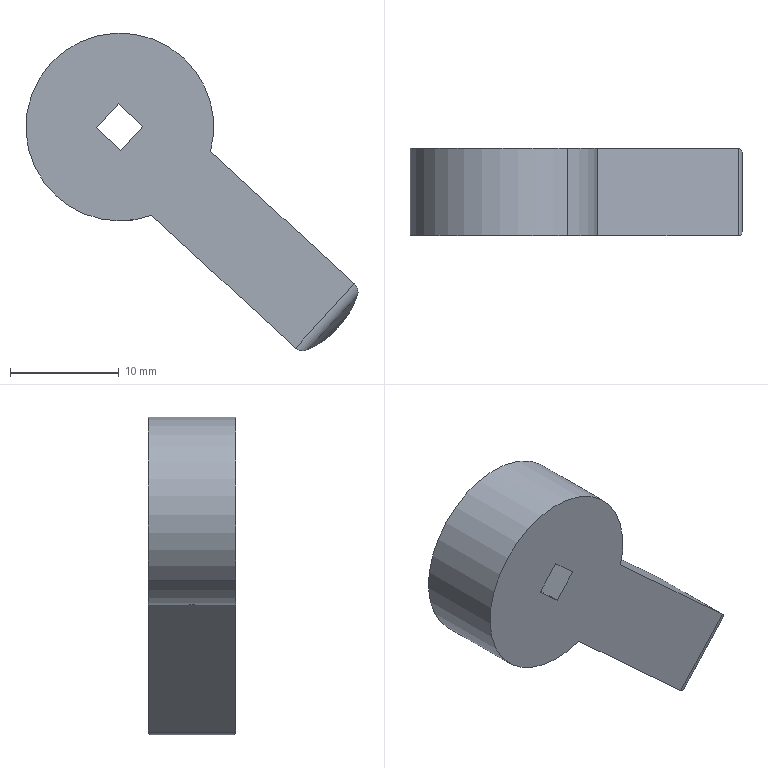Component | SolidWorks | Poussoir-1 | 1 solid | 24 faces | box 30.51 x 8 x 29.19 mm | volume 2976 mm3 | cylinder 11 | plane 9 | spline 4 | commonest cylinder face diameters 17 x4 2 x4 17.25 x3
STEP:
#1=CARTESIAN_POINT('',(2.86,2.961,-1.549));
#2=VERTEX_POINT('',#1);
#3=CARTESIAN_POINT('',(2.958,2.961,-1.887));
#4=VERTEX_POINT('',#3);
#5=CARTESIAN_POINT('',(2.63,2.961,-1.799));
#6=DIRECTION('',(0.,1.,-0.));
#7=DIRECTION('',(0.6774,0.,0.7356));
#8=AXIS2_PLACEMENT_3D('',#5,#6,#7);
#9=CIRCLE('',#8,0.3396);
#10=EDGE_CURVE('',#2,#4,#9,.T.);
#11=ORIENTED_EDGE('',*,*,#10,.F.);
#12=CARTESIAN_POINT('',(2.86,2.646,-1.549));
#13=VERTEX_POINT('',#12);
#14=CARTESIAN_POINT('',(2.86,2.961,-1.549));
#15=DIRECTION('',(-0.,-1.,0.));
#16=VECTOR('',#15,39.37);
#17=LINE('',#14,#16);
#18=EDGE_CURVE('',#2,#13,#17,.T.);
#19=ORIENTED_EDGE('',*,*,#18,.T.);
#20=CARTESIAN_POINT('',(2.958,2.646,-1.887));
#21=VERTEX_POINT('',#20);
#22=CARTESIAN_POINT('',(2.63,2.646,-1.799));
#23=DIRECTION('',(0.,1.,-0.));
#24=DIRECTION('',(0.6774,0.,0.7356));
#25=AXIS2_PLACEMENT_3D('',#22,#23,#24);
#26=CIRCLE('',#25,0.3396);
#27=EDGE_CURVE('',#13,#21,#26,.T.);
#28=ORIENTED_EDGE('',*,*,#27,.T.);
#29=CARTESIAN_POINT('',(2.958,2.961,-1.887));
#30=DIRECTION('',(-0.,-1.,0.));
#31=VECTOR('',#30,39.37);
#32=LINE('',#29,#31);
#33=EDGE_CURVE('',#4,#21,#32,.T.);
#34=ORIENTED_EDGE('',*,*,#33,.F.);
#35=EDGE_LOOP('',(#11,#19,#28,#34));
#36=FACE_OUTER_BOUND('',#35,.T.);
#37=CARTESIAN_POINT('',(2.63,2.961,-1.799));
#38=DIRECTION('',(-0.,-1.,0.));
#39=DIRECTION('',(-0.6774,0.,-0.7356));
#40=AXIS2_PLACEMENT_3D('',#37,#38,#39);
#41=CYLINDRICAL_SURFACE('',#40,0.3396);
#42=ADVANCED_FACE('',(#36),#41,.T.);
#43=ORIENTED_EDGE('',*,*,#18,.F.);
#44=CARTESIAN_POINT('',(2.4,2.961,-2.049));
#45=VERTEX_POINT('',#44);
#46=CARTESIAN_POINT('',(2.63,2.961,-1.799));
#47=DIRECTION('',(0.,1.,-0.));
#48=DIRECTION('',(0.6774,0.,0.7356));
#49=AXIS2_PLACEMENT_3D('',#46,#47,#48);
#50=CIRCLE('',#49,0.3396);
#51=EDGE_CURVE('',#45,#2,#50,.T.);
#52=ORIENTED_EDGE('',*,*,#51,.F.);
#53=CARTESIAN_POINT('',(2.4,2.646,-2.049));
#54=VERTEX_POINT('',#53);
#55=CARTESIAN_POINT('',(2.4,2.961,-2.049));
#56=DIRECTION('',(-0.,-1.,0.));
#57=VECTOR('',#56,39.37);
#58=LINE('',#55,#57);
#59=EDGE_CURVE('',#45,#54,#58,.T.);
#60=ORIENTED_EDGE('',*,*,#59,.T.);
#61=CARTESIAN_POINT('',(2.63,2.646,-1.799));
#62=DIRECTION('',(0.,1.,-0.));
#63=DIRECTION('',(0.6774,0.,0.7356));
#64=AXIS2_PLACEMENT_3D('',#61,#62,#63);
#65=CIRCLE('',#64,0.3396);
#66=EDGE_CURVE('',#54,#13,#65,.T.);
#67=ORIENTED_EDGE('',*,*,#66,.T.);
#68=EDGE_LOOP('',(#43,#52,#60,#67));
#69=FACE_OUTER_BOUND('',#68,.T.);
#70=CARTESIAN_POINT('',(2.63,2.961,-1.799));
#71=DIRECTION('',(-0.,-1.,0.));
#72=DIRECTION('',(-0.6774,0.,-0.7356));
#73=AXIS2_PLACEMENT_3D('',#70,#71,#72);
#74=CYLINDRICAL_SURFACE('',#73,0.3396);
#75=ADVANCED_FACE('',(#69),#74,.T.);
#76=CARTESIAN_POINT('',(3.419,2.803,-2.526));
#77=VERTEX_POINT('',#76);
#78=CARTESIAN_POINT('',(3.308,2.669,-2.605));
#79=VERTEX_POINT('',#78);
#80=CARTESIAN_POINT('',(3.419,2.803,-2.526));
#81=CARTESIAN_POINT('',(3.388,2.757,-2.56));
#82=CARTESIAN_POINT('',(3.35,2.712,-2.586));
#83=CARTESIAN_POINT('',(3.308,2.669,-2.605));
#84=(BOUNDED_CURVE()B_SPLINE_CURVE(3,(#80,#81,#82,#83),.UNSPECIFIED.,.F.,.F.)B_SPLINE_CURVE_WITH_KNOTS((4,4),(1.571,1.982),.UNSPECIFIED.)CURVE()GEOMETRIC_REPRESENTATION_ITEM()RATIONAL_B_SPLINE_CURVE((1.,0.9859,0.9859,1.))REPRESENTATION_ITEM(''));
#85=EDGE_CURVE('',#77,#79,#84,.T.);
#86=ORIENTED_EDGE('',*,*,#85,.T.);
#87=CARTESIAN_POINT('',(3.308,2.937,-2.605));
#88=VERTEX_POINT('',#87);
#89=CARTESIAN_POINT('',(3.308,2.646,-2.605));
#90=DIRECTION('',(0.,1.,-0.));
#91=VECTOR('',#90,39.37);
#92=LINE('',#89,#91);
#93=EDGE_CURVE('',#79,#88,#92,.T.);
#94=ORIENTED_EDGE('',*,*,#93,.T.);
#95=CARTESIAN_POINT('',(3.308,2.937,-2.605));
#96=CARTESIAN_POINT('',(3.35,2.895,-2.586));
#97=CARTESIAN_POINT('',(3.388,2.849,-2.56));
#98=CARTESIAN_POINT('',(3.419,2.803,-2.526));
#99=(BOUNDED_CURVE()B_SPLINE_CURVE(3,(#95,#96,#97,#98),.UNSPECIFIED.,.F.,.F.)B_SPLINE_CURVE_WITH_KNOTS((4,4),(1.159,1.571),.UNSPECIFIED.)CURVE()GEOMETRIC_REPRESENTATION_ITEM()RATIONAL_B_SPLINE_CURVE((1.,0.9859,0.9859,1.))REPRESENTATION_ITEM(''));
#100=EDGE_CURVE('',#88,#77,#99,.T.);
#101=ORIENTED_EDGE('',*,*,#100,.T.);
#102=EDGE_LOOP('',(#86,#94,#101));
#103=FACE_OUTER_BOUND('',#102,.T.);
#104=CARTESIAN_POINT('',(3.173,2.646,-2.299));
#105=DIRECTION('',(0.,1.,-0.));
#106=DIRECTION('',(0.6774,0.,0.7356));
#107=AXIS2_PLACEMENT_3D('',#104,#105,#106);
#108=CYLINDRICAL_SURFACE('',#107,0.3346);
#109=ADVANCED_FACE('',(#103),#108,.T.);
#110=CARTESIAN_POINT('',(3.479,2.961,-2.366));
#111=VERTEX_POINT('',#110);
#112=CARTESIAN_POINT('',(3.526,2.961,-2.41));
#113=DIRECTION('',(0.7356,-0.,-0.6774));
#114=VECTOR('',#113,39.37);
#115=LINE('',#112,#114);
#116=EDGE_CURVE('',#4,#111,#115,.T.);
#117=ORIENTED_EDGE('',*,*,#116,.T.);
#118=CARTESIAN_POINT('',(3.266,2.961,-2.598));
#119=VERTEX_POINT('',#118);
#120=CARTESIAN_POINT('',(3.266,2.961,-2.598));
#121=DIRECTION('',(-0.6774,0.,-0.7356));
#122=VECTOR('',#121,39.37);
#123=LINE('',#120,#122);
#124=EDGE_CURVE('',#111,#119,#123,.T.);
#125=ORIENTED_EDGE('',*,*,#124,.T.);
#126=CARTESIAN_POINT('',(2.745,2.961,-2.118));
#127=VERTEX_POINT('',#126);
#128=CARTESIAN_POINT('',(3.313,2.961,-2.641));
#129=DIRECTION('',(-0.7356,0.,0.6774));
#130=VECTOR('',#129,39.37);
#131=LINE('',#128,#130);
#132=EDGE_CURVE('',#119,#127,#131,.T.);
#133=ORIENTED_EDGE('',*,*,#132,.T.);
#134=CARTESIAN_POINT('',(2.63,2.961,-1.799));
#135=DIRECTION('',(0.,1.,-0.));
#136=DIRECTION('',(0.6774,0.,0.7356));
#137=AXIS2_PLACEMENT_3D('',#134,#135,#136);
#138=CIRCLE('',#137,0.3396);
#139=EDGE_CURVE('',#127,#45,#138,.T.);
#140=ORIENTED_EDGE('',*,*,#139,.T.);
#141=ORIENTED_EDGE('',*,*,#51,.T.);
#142=ORIENTED_EDGE('',*,*,#10,.T.);
#143=EDGE_LOOP('',(#117,#125,#133,#140,#141,#142));
#144=FACE_OUTER_BOUND('',#143,.T.);
#145=CARTESIAN_POINT('',(2.547,2.961,-1.802));
#146=VERTEX_POINT('',#145);
#147=CARTESIAN_POINT('',(2.627,2.961,-1.715));
#148=VERTEX_POINT('',#147);
#149=CARTESIAN_POINT('',(2.627,2.961,-1.715));
#150=DIRECTION('',(0.6774,-0.,0.7356));
#151=VECTOR('',#150,39.37);
#152=LINE('',#149,#151);
#153=EDGE_CURVE('',#146,#148,#152,.T.);
#154=ORIENTED_EDGE('',*,*,#153,.F.);
#155=CARTESIAN_POINT('',(2.634,2.961,-1.882));
#156=VERTEX_POINT('',#155);
#157=CARTESIAN_POINT('',(2.547,2.961,-1.802));
#158=DIRECTION('',(-0.7356,0.,0.6774));
#159=VECTOR('',#158,39.37);
#160=LINE('',#157,#159);
#161=EDGE_CURVE('',#156,#146,#160,.T.);
#162=ORIENTED_EDGE('',*,*,#161,.F.);
#163=CARTESIAN_POINT('',(2.714,2.961,-1.795));
#164=VERTEX_POINT('',#163);
#165=CARTESIAN_POINT('',(2.714,2.961,-1.795));
#166=DIRECTION('',(-0.6774,0.,-0.7356));
#167=VECTOR('',#166,39.37);
#168=LINE('',#165,#167);
#169=EDGE_CURVE('',#164,#156,#168,.T.);
#170=ORIENTED_EDGE('',*,*,#169,.F.);
#171=CARTESIAN_POINT('',(2.627,2.961,-1.715));
#172=DIRECTION('',(0.7356,-0.,-0.6774));
#173=VECTOR('',#172,39.37);
#174=LINE('',#171,#173);
#175=EDGE_CURVE('',#148,#164,#174,.T.);
#176=ORIENTED_EDGE('',*,*,#175,.F.);
#177=EDGE_LOOP('',(#154,#162,#170,#176));
#178=FACE_BOUND('',#177,.T.);
#179=CARTESIAN_POINT('',(2.63,2.961,-1.799));
#180=DIRECTION('',(0.,1.,-0.));
#181=DIRECTION('',(0.6774,-0.,0.7356));
#182=AXIS2_PLACEMENT_3D('',#179,#180,#181);
#183=PLANE('',#182);
#184=ADVANCED_FACE('',(#144,#178),#183,.T.);
#185=CARTESIAN_POINT('',(3.266,2.646,-2.598));
#186=VERTEX_POINT('',#185);
#187=CARTESIAN_POINT('',(2.745,2.646,-2.118));
#188=VERTEX_POINT('',#187);
#189=CARTESIAN_POINT('',(3.313,2.646,-2.641));
#190=DIRECTION('',(-0.7356,0.,0.6774));
#191=VECTOR('',#190,39.37);
#192=LINE('',#189,#191);
#193=EDGE_CURVE('',#186,#188,#192,.T.);
#194=ORIENTED_EDGE('',*,*,#193,.F.);
#195=CARTESIAN_POINT('',(3.479,2.646,-2.366));
#196=VERTEX_POINT('',#195);
#197=CARTESIAN_POINT('',(3.372,2.646,-2.482));
#198=DIRECTION('',(0.6774,-0.,0.7356));
#199=VECTOR('',#198,39.37);
#200=LINE('',#197,#199);
#201=EDGE_CURVE('',#186,#196,#200,.T.);
#202=ORIENTED_EDGE('',*,*,#201,.T.);
#203=CARTESIAN_POINT('',(3.526,2.646,-2.41));
#204=DIRECTION('',(0.7356,-0.,-0.6774));
#205=VECTOR('',#204,39.37);
#206=LINE('',#203,#205);
#207=EDGE_CURVE('',#21,#196,#206,.T.);
#208=ORIENTED_EDGE('',*,*,#207,.F.);
#209=ORIENTED_EDGE('',*,*,#27,.F.);
#210=ORIENTED_EDGE('',*,*,#66,.F.);
#211=CARTESIAN_POINT('',(2.63,2.646,-1.799));
#212=DIRECTION('',(0.,1.,-0.));
#213=DIRECTION('',(0.6774,0.,0.7356));
#214=AXIS2_PLACEMENT_3D('',#211,#212,#213);
#215=CIRCLE('',#214,0.3396);
#216=EDGE_CURVE('',#188,#54,#215,.T.);
#217=ORIENTED_EDGE('',*,*,#216,.F.);
#218=EDGE_LOOP('',(#194,#202,#208,#209,#210,#217));
#219=FACE_OUTER_BOUND('',#218,.T.);
#220=CARTESIAN_POINT('',(2.634,2.646,-1.882));
#221=VERTEX_POINT('',#220);
#222=CARTESIAN_POINT('',(2.547,2.646,-1.802));
#223=VERTEX_POINT('',#222);
#224=CARTESIAN_POINT('',(2.547,2.646,-1.802));
#225=DIRECTION('',(-0.7356,0.,0.6774));
#226=VECTOR('',#225,39.37);
#227=LINE('',#224,#226);
#228=EDGE_CURVE('',#221,#223,#227,.T.);
#229=ORIENTED_EDGE('',*,*,#228,.T.);
#230=CARTESIAN_POINT('',(2.627,2.646,-1.715));
#231=VERTEX_POINT('',#230);
#232=CARTESIAN_POINT('',(2.627,2.646,-1.715));
#233=DIRECTION('',(0.6774,-0.,0.7356));
#234=VECTOR('',#233,39.37);
#235=LINE('',#232,#234);
#236=EDGE_CURVE('',#223,#231,#235,.T.);
#237=ORIENTED_EDGE('',*,*,#236,.T.);
#238=CARTESIAN_POINT('',(2.714,2.646,-1.795));
#239=VERTEX_POINT('',#238);
#240=CARTESIAN_POINT('',(2.627,2.646,-1.715));
#241=DIRECTION('',(0.7356,-0.,-0.6774));
#242=VECTOR('',#241,39.37);
#243=LINE('',#240,#242);
#244=EDGE_CURVE('',#231,#239,#243,.T.);
#245=ORIENTED_EDGE('',*,*,#244,.T.);
#246=CARTESIAN_POINT('',(2.714,2.646,-1.795));
#247=DIRECTION('',(-0.6774,0.,-0.7356));
#248=VECTOR('',#247,39.37);
#249=LINE('',#246,#248);
#250=EDGE_CURVE('',#239,#221,#249,.T.);
#251=ORIENTED_EDGE('',*,*,#250,.T.);
#252=EDGE_LOOP('',(#229,#237,#245,#251));
#253=FACE_BOUND('',#252,.T.);
#254=CARTESIAN_POINT('',(2.63,2.646,-1.799));
#255=DIRECTION('',(0.,1.,-0.));
#256=DIRECTION('',(0.6774,-0.,0.7356));
#257=AXIS2_PLACEMENT_3D('',#254,#255,#256);
#258=PLANE('',#257);
#259=ADVANCED_FACE('',(#219,#253),#258,.F.);
#260=ORIENTED_EDGE('',*,*,#132,.F.);
#261=CARTESIAN_POINT('',(3.266,2.961,-2.598));
#262=DIRECTION('',(-0.,-1.,0.));
#263=VECTOR('',#262,39.37);
#264=LINE('',#261,#263);
#265=EDGE_CURVE('',#119,#186,#264,.T.);
#266=ORIENTED_EDGE('',*,*,#265,.T.);
#267=ORIENTED_EDGE('',*,*,#193,.T.);
#268=CARTESIAN_POINT('',(2.745,2.961,-2.118));
#269=DIRECTION('',(-0.,-1.,0.));
#270=VECTOR('',#269,39.37);
#271=LINE('',#268,#270);
#272=EDGE_CURVE('',#127,#188,#271,.T.);
#273=ORIENTED_EDGE('',*,*,#272,.F.);
#274=EDGE_LOOP('',(#260,#266,#267,#273));
#275=FACE_OUTER_BOUND('',#274,.T.);
#276=CARTESIAN_POINT('',(3.313,2.961,-2.641));
#277=DIRECTION('',(0.6774,-0.,0.7356));
#278=DIRECTION('',(0.7356,-0.,-0.6774));
#279=AXIS2_PLACEMENT_3D('',#276,#277,#278);
#280=PLANE('',#279);
#281=ADVANCED_FACE('',(#275),#280,.F.);
#282=ORIENTED_EDGE('',*,*,#59,.F.);
#283=ORIENTED_EDGE('',*,*,#139,.F.);
#284=ORIENTED_EDGE('',*,*,#272,.T.);
#285=ORIENTED_EDGE('',*,*,#216,.T.);
#286=EDGE_LOOP('',(#282,#283,#284,#285));
#287=FACE_OUTER_BOUND('',#286,.T.);
#288=CARTESIAN_POINT('',(2.605,2.803,-2.137));
#289=VERTEX_POINT('',#288);
#290=CARTESIAN_POINT('',(2.644,2.764,-2.138));
#291=VERTEX_POINT('',#290);
#292=CARTESIAN_POINT('',(2.605,2.803,-2.137));
#293=CARTESIAN_POINT('',(2.605,2.798,-2.137));
#294=CARTESIAN_POINT('',(2.606,2.793,-2.137));
#295=CARTESIAN_POINT('',(2.61,2.783,-2.138));
#296=CARTESIAN_POINT('',(2.613,2.779,-2.138));
#297=CARTESIAN_POINT('',(2.623,2.768,-2.138));
#298=CARTESIAN_POINT('',(2.634,2.764,-2.138));
#299=CARTESIAN_POINT('',(2.644,2.764,-2.138));
#300=B_SPLINE_CURVE_WITH_KNOTS('',3,(#292,#293,#294,#295,#296,#297,#298,#299),.UNSPECIFIED.,.F.,.F.,(4,2,2,4),(0.,0.0003909,0.0007817,0.001563),.UNSPECIFIED.);
#301=EDGE_CURVE('',#289,#291,#300,.T.);
#302=ORIENTED_EDGE('',*,*,#301,.T.);
#303=CARTESIAN_POINT('',(2.683,2.803,-2.134));
#304=VERTEX_POINT('',#303);
#305=CARTESIAN_POINT('',(2.644,2.764,-2.138));
#306=CARTESIAN_POINT('',(2.649,2.764,-2.138));
#307=CARTESIAN_POINT('',(2.654,2.765,-2.137));
#308=CARTESIAN_POINT('',(2.664,2.769,-2.137));
#309=CARTESIAN_POINT('',(2.668,2.772,-2.136));
#310=CARTESIAN_POINT('',(2.679,2.783,-2.135));
#311=CARTESIAN_POINT('',(2.683,2.793,-2.134));
#312=CARTESIAN_POINT('',(2.683,2.803,-2.134));
#313=B_SPLINE_CURVE_WITH_KNOTS('',3,(#305,#306,#307,#308,#309,#310,#311,#312),.UNSPECIFIED.,.F.,.F.,(4,2,2,4),(0.,0.0003909,0.0007817,0.001563),.UNSPECIFIED.);
#314=EDGE_CURVE('',#291,#304,#313,.T.);
#315=ORIENTED_EDGE('',*,*,#314,.T.);
#316=CARTESIAN_POINT('',(2.644,2.843,-2.138));
#317=VERTEX_POINT('',#316);
#318=CARTESIAN_POINT('',(2.683,2.803,-2.134));
#319=CARTESIAN_POINT('',(2.683,2.808,-2.134));
#320=CARTESIAN_POINT('',(2.682,2.813,-2.134));
#321=CARTESIAN_POINT('',(2.678,2.823,-2.135));
#322=CARTESIAN_POINT('',(2.675,2.827,-2.135));
#323=CARTESIAN_POINT('',(2.665,2.838,-2.137));
#324=CARTESIAN_POINT('',(2.654,2.843,-2.138));
#325=CARTESIAN_POINT('',(2.644,2.843,-2.138));
#326=B_SPLINE_CURVE_WITH_KNOTS('',3,(#318,#319,#320,#321,#322,#323,#324,#325),.UNSPECIFIED.,.F.,.F.,(4,2,2,4),(0.,0.0003909,0.0007817,0.001563),.UNSPECIFIED.);
#327=EDGE_CURVE('',#304,#317,#326,.T.);
#328=ORIENTED_EDGE('',*,*,#327,.T.);
#329=CARTESIAN_POINT('',(2.644,2.843,-2.138));
#330=CARTESIAN_POINT('',(2.639,2.843,-2.138));
#331=CARTESIAN_POINT('',(2.634,2.841,-2.138));
#332=CARTESIAN_POINT('',(2.624,2.838,-2.138));
#333=CARTESIAN_POINT('',(2.62,2.835,-2.138));
#334=CARTESIAN_POINT('',(2.609,2.824,-2.138));
#335=CARTESIAN_POINT('',(2.605,2.814,-2.137));
#336=CARTESIAN_POINT('',(2.605,2.803,-2.137));
#337=B_SPLINE_CURVE_WITH_KNOTS('',3,(#329,#330,#331,#332,#333,#334,#335,#336),.UNSPECIFIED.,.F.,.F.,(4,2,2,4),(0.,0.0003909,0.0007817,0.001563),.UNSPECIFIED.);
#338=EDGE_CURVE('',#317,#289,#337,.T.);
#339=ORIENTED_EDGE('',*,*,#338,.T.);
#340=EDGE_LOOP('',(#302,#315,#328,#339));
#341=FACE_BOUND('',#340,.T.);
#342=CARTESIAN_POINT('',(2.63,2.961,-1.799));
#343=DIRECTION('',(-0.,-1.,0.));
#344=DIRECTION('',(-0.6774,0.,-0.7356));
#345=AXIS2_PLACEMENT_3D('',#342,#343,#344);
#346=CYLINDRICAL_SURFACE('',#345,0.3396);
#347=ADVANCED_FACE('',(#287,#341),#346,.T.);
#348=ORIENTED_EDGE('',*,*,#207,.T.);
#349=CARTESIAN_POINT('',(3.479,2.961,-2.366));
#350=DIRECTION('',(0.,1.,-0.));
#351=VECTOR('',#350,39.37);
#352=LINE('',#349,#351);
#353=EDGE_CURVE('',#196,#111,#352,.T.);
#354=ORIENTED_EDGE('',*,*,#353,.T.);
#355=ORIENTED_EDGE('',*,*,#116,.F.);
#356=ORIENTED_EDGE('',*,*,#33,.T.);
#357=EDGE_LOOP('',(#348,#354,#355,#356));
#358=FACE_OUTER_BOUND('',#357,.T.);
#359=CARTESIAN_POINT('',(3.526,2.961,-2.41));
#360=DIRECTION('',(-0.6774,0.,-0.7356));
#361=DIRECTION('',(-0.7356,0.,0.6774));
#362=AXIS2_PLACEMENT_3D('',#359,#360,#361);
#363=PLANE('',#362);
#364=ADVANCED_FACE('',(#358),#363,.F.);
#365=ORIENTED_EDGE('',*,*,#228,.F.);
#366=CARTESIAN_POINT('',(2.634,2.961,-1.882));
#367=DIRECTION('',(-0.,-1.,0.));
#368=VECTOR('',#367,39.37);
#369=LINE('',#366,#368);
#370=EDGE_CURVE('',#156,#221,#369,.T.);
#371=ORIENTED_EDGE('',*,*,#370,.F.);
#372=ORIENTED_EDGE('',*,*,#161,.T.);
#373=CARTESIAN_POINT('',(2.547,2.961,-1.802));
#374=DIRECTION('',(-0.,-1.,0.));
#375=VECTOR('',#374,39.37);
#376=LINE('',#373,#375);
#377=EDGE_CURVE('',#146,#223,#376,.T.);
#378=ORIENTED_EDGE('',*,*,#377,.T.);
#379=EDGE_LOOP('',(#365,#371,#372,#378));
#380=FACE_OUTER_BOUND('',#379,.T.);
#381=CARTESIAN_POINT('',(2.547,2.961,-1.802));
#382=DIRECTION('',(0.6774,-0.,0.7356));
#383=DIRECTION('',(-0.,-1.,0.));
#384=AXIS2_PLACEMENT_3D('',#381,#382,#383);
#385=PLANE('',#384);
#386=ADVANCED_FACE('',(#380),#385,.T.);
#387=ORIENTED_EDGE('',*,*,#236,.F.);
#388=ORIENTED_EDGE('',*,*,#377,.F.);
#389=ORIENTED_EDGE('',*,*,#153,.T.);
#390=CARTESIAN_POINT('',(2.627,2.961,-1.715));
#391=DIRECTION('',(-0.,-1.,0.));
#392=VECTOR('',#391,39.37);
#393=LINE('',#390,#392);
#394=EDGE_CURVE('',#148,#231,#393,.T.);
#395=ORIENTED_EDGE('',*,*,#394,.T.);
#396=EDGE_LOOP('',(#387,#388,#389,#395));
#397=FACE_OUTER_BOUND('',#396,.T.);
#398=CARTESIAN_POINT('',(2.627,2.961,-1.715));
#399=DIRECTION('',(0.7356,-0.,-0.6774));
#400=DIRECTION('',(-0.6774,0.,-0.7356));
#401=AXIS2_PLACEMENT_3D('',#398,#399,#400);
#402=PLANE('',#401);
#403=ADVANCED_FACE('',(#397),#402,.T.);
#404=ORIENTED_EDGE('',*,*,#244,.F.);
#405=ORIENTED_EDGE('',*,*,#394,.F.);
#406=ORIENTED_EDGE('',*,*,#175,.T.);
#407=CARTESIAN_POINT('',(2.714,2.961,-1.795));
#408=DIRECTION('',(-0.,-1.,0.));
#409=VECTOR('',#408,39.37);
#410=LINE('',#407,#409);
#411=EDGE_CURVE('',#164,#239,#410,.T.);
#412=ORIENTED_EDGE('',*,*,#411,.T.);
#413=EDGE_LOOP('',(#404,#405,#406,#412));
#414=FACE_OUTER_BOUND('',#413,.T.);
#415=CARTESIAN_POINT('',(2.627,2.961,-1.715));
#416=DIRECTION('',(-0.6774,0.,-0.7356));
#417=DIRECTION('',(0.,1.,-0.));
#418=AXIS2_PLACEMENT_3D('',#415,#416,#417);
#419=PLANE('',#418);
#420=ADVANCED_FACE('',(#414),#419,.T.);
#421=ORIENTED_EDGE('',*,*,#250,.F.);
#422=ORIENTED_EDGE('',*,*,#411,.F.);
#423=ORIENTED_EDGE('',*,*,#169,.T.);
#424=ORIENTED_EDGE('',*,*,#370,.T.);
#425=EDGE_LOOP('',(#421,#422,#423,#424));
#426=FACE_OUTER_BOUND('',#425,.T.);
#427=CARTESIAN_POINT('',(2.714,2.961,-1.795));
#428=DIRECTION('',(-0.7356,0.,0.6774));
#429=DIRECTION('',(0.6774,-0.,0.7356));
#430=AXIS2_PLACEMENT_3D('',#427,#428,#429);
#431=PLANE('',#430);
#432=ADVANCED_FACE('',(#426),#431,.T.);
#433=CARTESIAN_POINT('',(3.489,2.937,-2.408));
#434=VERTEX_POINT('',#433);
#435=CARTESIAN_POINT('',(3.419,2.803,-2.526));
#436=CARTESIAN_POINT('',(3.451,2.849,-2.492));
#437=CARTESIAN_POINT('',(3.474,2.895,-2.452));
#438=CARTESIAN_POINT('',(3.489,2.937,-2.408));
#439=(BOUNDED_CURVE()B_SPLINE_CURVE(3,(#435,#436,#437,#438),.UNSPECIFIED.,.F.,.F.)B_SPLINE_CURVE_WITH_KNOTS((4,4),(4.712,5.124),.UNSPECIFIED.)CURVE()GEOMETRIC_REPRESENTATION_ITEM()RATIONAL_B_SPLINE_CURVE((1.,0.9859,0.9859,1.))REPRESENTATION_ITEM(''));
#440=EDGE_CURVE('',#77,#434,#439,.T.);
#441=ORIENTED_EDGE('',*,*,#440,.T.);
#442=CARTESIAN_POINT('',(3.489,2.669,-2.408));
#443=VERTEX_POINT('',#442);
#444=CARTESIAN_POINT('',(3.489,2.646,-2.408));
#445=DIRECTION('',(-0.,-1.,0.));
#446=VECTOR('',#445,39.37);
#447=LINE('',#444,#446);
#448=EDGE_CURVE('',#434,#443,#447,.T.);
#449=ORIENTED_EDGE('',*,*,#448,.T.);
#450=CARTESIAN_POINT('',(3.489,2.669,-2.408));
#451=CARTESIAN_POINT('',(3.474,2.712,-2.452));
#452=CARTESIAN_POINT('',(3.451,2.757,-2.492));
#453=CARTESIAN_POINT('',(3.419,2.803,-2.526));
#454=(BOUNDED_CURVE()B_SPLINE_CURVE(3,(#450,#451,#452,#453),.UNSPECIFIED.,.F.,.F.)B_SPLINE_CURVE_WITH_KNOTS((4,4),(4.301,4.712),.UNSPECIFIED.)CURVE()GEOMETRIC_REPRESENTATION_ITEM()RATIONAL_B_SPLINE_CURVE((1.,0.9859,0.9859,1.))REPRESENTATION_ITEM(''));
#455=EDGE_CURVE('',#443,#77,#454,.T.);
#456=ORIENTED_EDGE('',*,*,#455,.T.);
#457=EDGE_LOOP('',(#441,#449,#456));
#458=FACE_OUTER_BOUND('',#457,.T.);
#459=CARTESIAN_POINT('',(3.173,2.646,-2.299));
#460=DIRECTION('',(0.,1.,-0.));
#461=DIRECTION('',(0.6774,0.,0.7356));
#462=AXIS2_PLACEMENT_3D('',#459,#460,#461);
#463=CYLINDRICAL_SURFACE('',#462,0.3346);
#464=ADVANCED_FACE('',(#458),#463,.T.);
#465=ORIENTED_EDGE('',*,*,#100,.F.);
#466=CARTESIAN_POINT('',(3.505,2.937,-2.391));
#467=DIRECTION('',(0.6774,-0.,0.7356));
#468=VECTOR('',#467,39.37);
#469=LINE('',#466,#468);
#470=EDGE_CURVE('',#88,#434,#469,.T.);
#471=ORIENTED_EDGE('',*,*,#470,.T.);
#472=ORIENTED_EDGE('',*,*,#440,.F.);
#473=EDGE_LOOP('',(#465,#471,#472));
#474=FACE_OUTER_BOUND('',#473,.T.);
#475=CARTESIAN_POINT('',(3.28,2.803,-2.183));
#476=DIRECTION('',(-0.6774,0.,-0.7356));
#477=DIRECTION('',(-0.7356,0.,0.6774));
#478=AXIS2_PLACEMENT_3D('',#475,#476,#477);
#479=CYLINDRICAL_SURFACE('',#478,0.3346);
#480=ADVANCED_FACE('',(#474),#479,.T.);
#481=ORIENTED_EDGE('',*,*,#455,.F.);
#482=CARTESIAN_POINT('',(3.505,2.669,-2.391));
#483=DIRECTION('',(-0.6774,0.,-0.7356));
#484=VECTOR('',#483,39.37);
#485=LINE('',#482,#484);
#486=EDGE_CURVE('',#443,#79,#485,.T.);
#487=ORIENTED_EDGE('',*,*,#486,.T.);
#488=ORIENTED_EDGE('',*,*,#85,.F.);
#489=EDGE_LOOP('',(#481,#487,#488));
#490=FACE_OUTER_BOUND('',#489,.T.);
#491=CARTESIAN_POINT('',(3.28,2.803,-2.183));
#492=DIRECTION('',(-0.6774,0.,-0.7356));
#493=DIRECTION('',(-0.7356,0.,0.6774));
#494=AXIS2_PLACEMENT_3D('',#491,#492,#493);
#495=CYLINDRICAL_SURFACE('',#494,0.3346);
#496=ADVANCED_FACE('',(#490),#495,.T.);
#497=CARTESIAN_POINT('',(3.308,2.669,-2.605));
#498=CARTESIAN_POINT('',(3.293,2.654,-2.612));
#499=CARTESIAN_POINT('',(3.277,2.646,-2.609));
#500=CARTESIAN_POINT('',(3.266,2.646,-2.598));
#501=(BOUNDED_CURVE()B_SPLINE_CURVE(3,(#497,#498,#499,#500),.UNSPECIFIED.,.F.,.F.)B_SPLINE_CURVE_WITH_KNOTS((4,4),(1.982,3.142),.UNSPECIFIED.)CURVE()GEOMETRIC_REPRESENTATION_ITEM()RATIONAL_B_SPLINE_CURVE((1.,0.8911,0.8911,1.))REPRESENTATION_ITEM(''));
#502=EDGE_CURVE('',#79,#186,#501,.T.);
#503=ORIENTED_EDGE('',*,*,#502,.F.);
#504=ORIENTED_EDGE('',*,*,#486,.F.);
#505=CARTESIAN_POINT('',(3.479,2.646,-2.366));
#506=CARTESIAN_POINT('',(3.491,2.646,-2.377));
#507=CARTESIAN_POINT('',(3.495,2.654,-2.393));
#508=CARTESIAN_POINT('',(3.489,2.669,-2.408));
#509=(BOUNDED_CURVE()B_SPLINE_CURVE(3,(#505,#506,#507,#508),.UNSPECIFIED.,.F.,.F.)B_SPLINE_CURVE_WITH_KNOTS((4,4),(3.142,4.301),.UNSPECIFIED.)CURVE()GEOMETRIC_REPRESENTATION_ITEM()RATIONAL_B_SPLINE_CURVE((1.,0.8911,0.8911,1.))REPRESENTATION_ITEM(''));
#510=EDGE_CURVE('',#196,#443,#509,.T.);
#511=ORIENTED_EDGE('',*,*,#510,.F.);
#512=ORIENTED_EDGE('',*,*,#201,.F.);
#513=EDGE_LOOP('',(#503,#504,#511,#512));
#514=FACE_OUTER_BOUND('',#513,.T.);
#515=CARTESIAN_POINT('',(3.479,2.685,-2.366));
#516=DIRECTION('',(-0.6774,0.,-0.7356));
#517=DIRECTION('',(-0.7356,0.,0.6774));
#518=AXIS2_PLACEMENT_3D('',#515,#516,#517);
#519=CYLINDRICAL_SURFACE('',#518,0.03937);
#520=ADVANCED_FACE('',(#514),#519,.T.);
#521=ORIENTED_EDGE('',*,*,#510,.T.);
#522=ORIENTED_EDGE('',*,*,#448,.F.);
#523=CARTESIAN_POINT('',(3.479,2.961,-2.366));
#524=CARTESIAN_POINT('',(3.491,2.961,-2.377));
#525=CARTESIAN_POINT('',(3.495,2.952,-2.393));
#526=CARTESIAN_POINT('',(3.489,2.937,-2.408));
#527=(BOUNDED_CURVE()B_SPLINE_CURVE(3,(#523,#524,#525,#526),.UNSPECIFIED.,.F.,.F.)B_SPLINE_CURVE_WITH_KNOTS((4,4),(0.,1.159),.UNSPECIFIED.)CURVE()GEOMETRIC_REPRESENTATION_ITEM()RATIONAL_B_SPLINE_CURVE((1.,0.8911,0.8911,1.))REPRESENTATION_ITEM(''));
#528=EDGE_CURVE('',#111,#434,#527,.T.);
#529=ORIENTED_EDGE('',*,*,#528,.F.);
#530=ORIENTED_EDGE('',*,*,#353,.F.);
#531=EDGE_LOOP('',(#521,#522,#529,#530));
#532=FACE_OUTER_BOUND('',#531,.T.);
#533=CARTESIAN_POINT('',(3.452,2.646,-2.395));
#534=DIRECTION('',(0.,1.,-0.));
#535=DIRECTION('',(0.6774,0.,0.7356));
#536=AXIS2_PLACEMENT_3D('',#533,#534,#535);
#537=CYLINDRICAL_SURFACE('',#536,0.03937);
#538=ADVANCED_FACE('',(#532),#537,.T.);
#539=ORIENTED_EDGE('',*,*,#502,.T.);
#540=ORIENTED_EDGE('',*,*,#265,.F.);
#541=CARTESIAN_POINT('',(3.308,2.937,-2.605));
#542=CARTESIAN_POINT('',(3.293,2.952,-2.612));
#543=CARTESIAN_POINT('',(3.277,2.961,-2.609));
#544=CARTESIAN_POINT('',(3.266,2.961,-2.598));
#545=(BOUNDED_CURVE()B_SPLINE_CURVE(3,(#541,#542,#543,#544),.UNSPECIFIED.,.F.,.F.)B_SPLINE_CURVE_WITH_KNOTS((4,4),(5.124,6.283),.UNSPECIFIED.)CURVE()GEOMETRIC_REPRESENTATION_ITEM()RATIONAL_B_SPLINE_CURVE((1.,0.8911,0.8911,1.))REPRESENTATION_ITEM(''));
#546=EDGE_CURVE('',#88,#119,#545,.T.);
#547=ORIENTED_EDGE('',*,*,#546,.F.);
#548=ORIENTED_EDGE('',*,*,#93,.F.);
#549=EDGE_LOOP('',(#539,#540,#547,#548));
#550=FACE_OUTER_BOUND('',#549,.T.);
#551=CARTESIAN_POINT('',(3.292,2.646,-2.569));
#552=DIRECTION('',(0.,1.,-0.));
#553=DIRECTION('',(0.6774,0.,0.7356));
#554=AXIS2_PLACEMENT_3D('',#551,#552,#553);
#555=CYLINDRICAL_SURFACE('',#554,0.03937);
#556=ADVANCED_FACE('',(#550),#555,.T.);
#557=ORIENTED_EDGE('',*,*,#528,.T.);
#558=ORIENTED_EDGE('',*,*,#470,.F.);
#559=ORIENTED_EDGE('',*,*,#546,.T.);
#560=ORIENTED_EDGE('',*,*,#124,.F.);
#561=EDGE_LOOP('',(#557,#558,#559,#560));
#562=FACE_OUTER_BOUND('',#561,.T.);
#563=CARTESIAN_POINT('',(3.479,2.921,-2.366));
#564=DIRECTION('',(-0.6774,0.,-0.7356));
#565=DIRECTION('',(-0.7356,0.,0.6774));
#566=AXIS2_PLACEMENT_3D('',#563,#564,#565);
#567=CYLINDRICAL_SURFACE('',#566,0.03937);
#568=ADVANCED_FACE('',(#562),#567,.T.);
#569=CARTESIAN_POINT('',(2.637,2.803,-2.119));
#570=VERTEX_POINT('',#569);
#571=CARTESIAN_POINT('',(2.643,2.808,-2.118));
#572=VERTEX_POINT('',#571);
#573=CARTESIAN_POINT('',(2.637,2.803,-2.119));
#574=CARTESIAN_POINT('',(2.637,2.805,-2.119));
#575=CARTESIAN_POINT('',(2.638,2.806,-2.119));
#576=CARTESIAN_POINT('',(2.64,2.808,-2.118));
#577=CARTESIAN_POINT('',(2.642,2.808,-2.118));
#578=CARTESIAN_POINT('',(2.643,2.808,-2.118));
#579=B_SPLINE_CURVE_WITH_KNOTS('',3,(#573,#574,#575,#576,#577,#578),.UNSPECIFIED.,.F.,.F.,(4,2,4),(0.,0.0001202,0.0002403),.UNSPECIFIED.);
#580=EDGE_CURVE('',#570,#572,#579,.T.);
#581=ORIENTED_EDGE('',*,*,#580,.T.);
#582=CARTESIAN_POINT('',(2.65,2.803,-2.118));
#583=VERTEX_POINT('',#582);
#584=CARTESIAN_POINT('',(2.643,2.808,-2.118));
#585=CARTESIAN_POINT('',(2.644,2.808,-2.118));
#586=CARTESIAN_POINT('',(2.645,2.808,-2.118));
#587=CARTESIAN_POINT('',(2.645,2.808,-2.118));
#588=CARTESIAN_POINT('',(2.646,2.808,-2.118));
#589=CARTESIAN_POINT('',(2.646,2.808,-2.118));
#590=CARTESIAN_POINT('',(2.647,2.808,-2.118));
#591=CARTESIAN_POINT('',(2.647,2.807,-2.118));
#592=CARTESIAN_POINT('',(2.648,2.807,-2.118));
#593=CARTESIAN_POINT('',(2.648,2.807,-2.118));
#594=CARTESIAN_POINT('',(2.649,2.806,-2.118));
#595=CARTESIAN_POINT('',(2.649,2.806,-2.118));
#596=CARTESIAN_POINT('',(2.649,2.805,-2.118));
#597=CARTESIAN_POINT('',(2.65,2.805,-2.118));
#598=CARTESIAN_POINT('',(2.65,2.804,-2.118));
#599=CARTESIAN_POINT('',(2.65,2.804,-2.118));
#600=CARTESIAN_POINT('',(2.65,2.804,-2.118));
#601=CARTESIAN_POINT('',(2.65,2.803,-2.118));
#602=CARTESIAN_POINT('',(2.65,2.803,-2.118));
#603=B_SPLINE_CURVE_WITH_KNOTS('',3,(#584,#585,#586,#587,#588,#589,#590,#591,#592,#593,#594,#595,#596,#597,#598,#599,#600,#601,#602),.UNSPECIFIED.,.F.,.F.,(4,3,3,3,3,3,4),(0.,0.00005334,0.00008948,0.0001358,0.0001824,0.0002188,0.0002379),.UNSPECIFIED.);
#604=EDGE_CURVE('',#572,#583,#603,.T.);
#605=ORIENTED_EDGE('',*,*,#604,.T.);
#606=CARTESIAN_POINT('',(2.643,2.798,-2.118));
#607=VERTEX_POINT('',#606);
#608=CARTESIAN_POINT('',(2.65,2.803,-2.118));
#609=CARTESIAN_POINT('',(2.65,2.802,-2.118));
#610=CARTESIAN_POINT('',(2.649,2.8,-2.118));
#611=CARTESIAN_POINT('',(2.646,2.798,-2.118));
#612=CARTESIAN_POINT('',(2.645,2.798,-2.118));
#613=CARTESIAN_POINT('',(2.643,2.798,-2.118));
#614=B_SPLINE_CURVE_WITH_KNOTS('',3,(#608,#609,#610,#611,#612,#613),.UNSPECIFIED.,.F.,.F.,(4,2,4),(0.,0.0001202,0.0002403),.UNSPECIFIED.);
#615=EDGE_CURVE('',#583,#607,#614,.T.);
#616=ORIENTED_EDGE('',*,*,#615,.T.);
#617=CARTESIAN_POINT('',(2.643,2.798,-2.118));
#618=CARTESIAN_POINT('',(2.643,2.798,-2.118));
#619=CARTESIAN_POINT('',(2.642,2.798,-2.118));
#620=CARTESIAN_POINT('',(2.641,2.798,-2.118));
#621=CARTESIAN_POINT('',(2.641,2.798,-2.118));
#622=CARTESIAN_POINT('',(2.64,2.798,-2.118));
#623=CARTESIAN_POINT('',(2.64,2.799,-2.119));
#624=CARTESIAN_POINT('',(2.639,2.799,-2.119));
#625=CARTESIAN_POINT('',(2.639,2.799,-2.119));
#626=CARTESIAN_POINT('',(2.638,2.8,-2.119));
#627=CARTESIAN_POINT('',(2.638,2.8,-2.119));
#628=CARTESIAN_POINT('',(2.637,2.801,-2.119));
#629=CARTESIAN_POINT('',(2.637,2.801,-2.119));
#630=CARTESIAN_POINT('',(2.637,2.801,-2.119));
#631=CARTESIAN_POINT('',(2.637,2.802,-2.119));
#632=CARTESIAN_POINT('',(2.637,2.802,-2.119));
#633=CARTESIAN_POINT('',(2.637,2.803,-2.119));
#634=CARTESIAN_POINT('',(2.637,2.803,-2.119));
#635=CARTESIAN_POINT('',(2.637,2.803,-2.119));
#636=B_SPLINE_CURVE_WITH_KNOTS('',3,(#617,#618,#619,#620,#621,#622,#623,#624,#625,#626,#627,#628,#629,#630,#631,#632,#633,#634,#635),.UNSPECIFIED.,.F.,.F.,(4,3,3,3,3,3,4),(0.,0.00005334,0.00008948,0.0001358,0.0001824,0.0002188,0.0002379),.UNSPECIFIED.);
#637=EDGE_CURVE('',#607,#570,#636,.T.);
#638=ORIENTED_EDGE('',*,*,#637,.T.);
#639=EDGE_LOOP('',(#581,#605,#616,#638));
#640=FACE_OUTER_BOUND('',#639,.T.);
#641=CARTESIAN_POINT('',(2.604,2.764,-2.12));
#642=DIRECTION('',(-0.0411,0.,0.9992));
#643=DIRECTION('',(0.9992,-0.,0.0411));
#644=AXIS2_PLACEMENT_3D('',#641,#642,#643);
#645=PLANE('',#644);
#646=ADVANCED_FACE('',(#640),#645,.F.);
#647=CARTESIAN_POINT('',(2.645,2.798,-2.158));
#648=DIRECTION('',(-0.9992,0.,-0.0411));
#649=DIRECTION('',(0.0411,0.,-0.9992));
#650=AXIS2_PLACEMENT_3D('',#647,#648,#649);
#651=CIRCLE('',#650,0.03937);
#652=EDGE_CURVE('',#291,#607,#651,.T.);
#653=ORIENTED_EDGE('',*,*,#652,.F.);
#654=ORIENTED_EDGE('',*,*,#301,.F.);
#655=CARTESIAN_POINT('',(2.638,2.803,-2.158));
#656=DIRECTION('',(0.,-1.,0.));
#657=DIRECTION('',(-0.6774,0.,-0.7356));
#658=AXIS2_PLACEMENT_3D('',#655,#656,#657);
#659=CIRCLE('',#658,0.03937);
#660=EDGE_CURVE('',#570,#289,#659,.T.);
#661=ORIENTED_EDGE('',*,*,#660,.F.);
#662=ORIENTED_EDGE('',*,*,#637,.F.);
#663=EDGE_LOOP('',(#653,#654,#661,#662));
#664=FACE_OUTER_BOUND('',#663,.T.);
#665=CARTESIAN_POINT('',(2.643,2.798,-2.118));
#666=CARTESIAN_POINT('',(2.643,2.775,-2.118));
#667=CARTESIAN_POINT('',(2.644,2.764,-2.138));
#668=CARTESIAN_POINT('',(2.642,2.798,-2.118));
#669=CARTESIAN_POINT('',(2.637,2.775,-2.119));
#670=CARTESIAN_POINT('',(2.636,2.764,-2.138));
#671=CARTESIAN_POINT('',(2.64,2.798,-2.118));
#672=CARTESIAN_POINT('',(2.631,2.777,-2.119));
#673=CARTESIAN_POINT('',(2.628,2.766,-2.138));
#674=CARTESIAN_POINT('',(2.638,2.8,-2.119));
#675=CARTESIAN_POINT('',(2.624,2.783,-2.119));
#676=CARTESIAN_POINT('',(2.616,2.775,-2.138));
#677=CARTESIAN_POINT('',(2.638,2.8,-2.119));
#678=CARTESIAN_POINT('',(2.621,2.786,-2.119));
#679=CARTESIAN_POINT('',(2.613,2.778,-2.138));
#680=CARTESIAN_POINT('',(2.637,2.801,-2.119));
#681=CARTESIAN_POINT('',(2.618,2.791,-2.119));
#682=CARTESIAN_POINT('',(2.608,2.786,-2.138));
#683=CARTESIAN_POINT('',(2.637,2.802,-2.119));
#684=CARTESIAN_POINT('',(2.617,2.794,-2.119));
#685=CARTESIAN_POINT('',(2.607,2.789,-2.138));
#686=CARTESIAN_POINT('',(2.637,2.802,-2.119));
#687=CARTESIAN_POINT('',(2.616,2.798,-2.119));
#688=CARTESIAN_POINT('',(2.605,2.796,-2.137));
#689=CARTESIAN_POINT('',(2.637,2.803,-2.119));
#690=CARTESIAN_POINT('',(2.616,2.801,-2.119));
#691=CARTESIAN_POINT('',(2.605,2.799,-2.137));
#692=CARTESIAN_POINT('',(2.637,2.803,-2.119));
#693=CARTESIAN_POINT('',(2.616,2.803,-2.119));
#694=CARTESIAN_POINT('',(2.605,2.803,-2.137));
#695=(BOUNDED_SURFACE()B_SPLINE_SURFACE(3,2,((#665,#666,#667),(#668,#669,#670),(#671,#672,#673),(#674,#675,#676),(#677,#678,#679),(#680,#681,#682),(#683,#684,#685),(#686,#687,#688),(#689,#690,#691),(#692,#693,#694)),.UNSPECIFIED.,.F.,.F.,.F.)B_SPLINE_SURFACE_WITH_KNOTS((4,2,2,2,4),(3,3),(0.0004347,0.0005529,0.0006121,0.0006416,0.0006712),(0.,1.),.UNSPECIFIED.)GEOMETRIC_REPRESENTATION_ITEM()RATIONAL_B_SPLINE_SURFACE(((1.,0.866,1.),(1.,0.866,1.),(1.,0.8683,1.),(1.,0.8741,1.),(1.,0.8764,1.),(1.,0.8796,1.),(1.,0.8807,1.),(1.,0.8822,1.),(1.,0.8827,1.),(1.,0.8827,1.)))REPRESENTATION_ITEM('')SURFACE());
#696=ADVANCED_FACE('',(#664),#695,.F.);
#697=ORIENTED_EDGE('',*,*,#660,.T.);
#698=ORIENTED_EDGE('',*,*,#338,.F.);
#699=CARTESIAN_POINT('',(2.645,2.808,-2.158));
#700=DIRECTION('',(-0.9992,-0.,-0.0411));
#701=DIRECTION('',(-0.0411,0.,0.9992));
#702=AXIS2_PLACEMENT_3D('',#699,#700,#701);
#703=CIRCLE('',#702,0.03937);
#704=EDGE_CURVE('',#572,#317,#703,.T.);
#705=ORIENTED_EDGE('',*,*,#704,.F.);
#706=ORIENTED_EDGE('',*,*,#580,.F.);
#707=EDGE_LOOP('',(#697,#698,#705,#706));
#708=FACE_OUTER_BOUND('',#707,.T.);
#709=CARTESIAN_POINT('',(2.637,2.803,-2.119));
#710=CARTESIAN_POINT('',(2.616,2.803,-2.119));
#711=CARTESIAN_POINT('',(2.605,2.803,-2.137));
#712=CARTESIAN_POINT('',(2.637,2.804,-2.119));
#713=CARTESIAN_POINT('',(2.616,2.806,-2.119));
#714=CARTESIAN_POINT('',(2.605,2.807,-2.137));
#715=CARTESIAN_POINT('',(2.637,2.804,-2.119));
#716=CARTESIAN_POINT('',(2.616,2.808,-2.119));
#717=CARTESIAN_POINT('',(2.605,2.811,-2.137));
#718=CARTESIAN_POINT('',(2.637,2.805,-2.119));
#719=CARTESIAN_POINT('',(2.617,2.813,-2.119));
#720=CARTESIAN_POINT('',(2.607,2.817,-2.138));
#721=CARTESIAN_POINT('',(2.637,2.805,-2.119));
#722=CARTESIAN_POINT('',(2.618,2.815,-2.119));
#723=CARTESIAN_POINT('',(2.608,2.82,-2.138));
#724=CARTESIAN_POINT('',(2.638,2.806,-2.119));
#725=CARTESIAN_POINT('',(2.621,2.82,-2.119));
#726=CARTESIAN_POINT('',(2.613,2.828,-2.138));
#727=CARTESIAN_POINT('',(2.638,2.807,-2.119));
#728=CARTESIAN_POINT('',(2.624,2.823,-2.119));
#729=CARTESIAN_POINT('',(2.617,2.832,-2.138));
#730=CARTESIAN_POINT('',(2.64,2.808,-2.118));
#731=CARTESIAN_POINT('',(2.631,2.829,-2.119));
#732=CARTESIAN_POINT('',(2.628,2.84,-2.138));
#733=CARTESIAN_POINT('',(2.642,2.808,-2.118));
#734=CARTESIAN_POINT('',(2.637,2.831,-2.119));
#735=CARTESIAN_POINT('',(2.636,2.843,-2.138));
#736=CARTESIAN_POINT('',(2.643,2.808,-2.118));
#737=CARTESIAN_POINT('',(2.643,2.831,-2.118));
#738=CARTESIAN_POINT('',(2.644,2.843,-2.138));
#739=(BOUNDED_SURFACE()B_SPLINE_SURFACE(3,2,((#709,#710,#711),(#712,#713,#714),(#715,#716,#717),(#718,#719,#720),(#721,#722,#723),(#724,#725,#726),(#727,#728,#729),(#730,#731,#732),(#733,#734,#735),(#736,#737,#738)),.UNSPECIFIED.,.F.,.F.,.F.)B_SPLINE_SURFACE_WITH_KNOTS((4,2,2,2,4),(3,3),(0.0003492,0.000379,0.0004087,0.0004682,0.0005871),(0.,1.),.UNSPECIFIED.)GEOMETRIC_REPRESENTATION_ITEM()RATIONAL_B_SPLINE_SURFACE(((1.,0.8827,1.),(1.,0.8827,1.),(1.,0.8822,1.),(1.,0.8807,1.),(1.,0.8796,1.),(1.,0.8764,1.),(1.,0.874,1.),(1.,0.8683,1.),(1.,0.866,1.),(1.,0.866,1.)))REPRESENTATION_ITEM('')SURFACE());
#740=ADVANCED_FACE('',(#708),#739,.F.);
#741=ORIENTED_EDGE('',*,*,#652,.T.);
#742=ORIENTED_EDGE('',*,*,#615,.F.);
#743=CARTESIAN_POINT('',(2.652,2.803,-2.157));
#744=DIRECTION('',(0.,-1.,0.));
#745=DIRECTION('',(0.6774,0.,0.7356));
#746=AXIS2_PLACEMENT_3D('',#743,#744,#745);
#747=CIRCLE('',#746,0.03937);
#748=EDGE_CURVE('',#304,#583,#747,.T.);
#749=ORIENTED_EDGE('',*,*,#748,.F.);
#750=ORIENTED_EDGE('',*,*,#314,.F.);
#751=EDGE_LOOP('',(#741,#742,#749,#750));
#752=FACE_OUTER_BOUND('',#751,.T.);
#753=CARTESIAN_POINT('',(2.65,2.803,-2.118));
#754=CARTESIAN_POINT('',(2.671,2.803,-2.117));
#755=CARTESIAN_POINT('',(2.683,2.803,-2.134));
#756=CARTESIAN_POINT('',(2.65,2.803,-2.118));
#757=CARTESIAN_POINT('',(2.671,2.801,-2.117));
#758=CARTESIAN_POINT('',(2.683,2.799,-2.134));
#759=CARTESIAN_POINT('',(2.65,2.802,-2.118));
#760=CARTESIAN_POINT('',(2.671,2.798,-2.117));
#761=CARTESIAN_POINT('',(2.683,2.796,-2.134));
#762=CARTESIAN_POINT('',(2.65,2.802,-2.118));
#763=CARTESIAN_POINT('',(2.669,2.794,-2.117));
#764=CARTESIAN_POINT('',(2.681,2.789,-2.135));
#765=CARTESIAN_POINT('',(2.65,2.801,-2.118));
#766=CARTESIAN_POINT('',(2.668,2.791,-2.117));
#767=CARTESIAN_POINT('',(2.68,2.786,-2.135));
#768=CARTESIAN_POINT('',(2.649,2.8,-2.118));
#769=CARTESIAN_POINT('',(2.666,2.786,-2.117));
#770=CARTESIAN_POINT('',(2.675,2.778,-2.135));
#771=CARTESIAN_POINT('',(2.648,2.8,-2.118));
#772=CARTESIAN_POINT('',(2.663,2.783,-2.118));
#773=CARTESIAN_POINT('',(2.672,2.775,-2.136));
#774=CARTESIAN_POINT('',(2.646,2.798,-2.118));
#775=CARTESIAN_POINT('',(2.655,2.777,-2.118));
#776=CARTESIAN_POINT('',(2.66,2.766,-2.137));
#777=CARTESIAN_POINT('',(2.645,2.798,-2.118));
#778=CARTESIAN_POINT('',(2.649,2.775,-2.118));
#779=CARTESIAN_POINT('',(2.652,2.764,-2.138));
#780=CARTESIAN_POINT('',(2.643,2.798,-2.118));
#781=CARTESIAN_POINT('',(2.643,2.775,-2.118));
#782=CARTESIAN_POINT('',(2.644,2.764,-2.138));
#783=(BOUNDED_SURFACE()B_SPLINE_SURFACE(3,2,((#753,#754,#755),(#756,#757,#758),(#759,#760,#761),(#762,#763,#764),(#765,#766,#767),(#768,#769,#770),(#771,#772,#773),(#774,#775,#776),(#777,#778,#779),(#780,#781,#782)),.UNSPECIFIED.,.F.,.F.,.F.)B_SPLINE_SURFACE_WITH_KNOTS((4,2,2,2,4),(3,3),(0.0003492,0.000379,0.0004087,0.0004682,0.0005871),(0.,1.),.UNSPECIFIED.)GEOMETRIC_REPRESENTATION_ITEM()RATIONAL_B_SPLINE_SURFACE(((1.,0.8827,1.),(1.,0.8827,1.),(1.,0.8822,1.),(1.,0.8807,1.),(1.,0.8796,1.),(1.,0.8764,1.),(1.,0.874,1.),(1.,0.8683,1.),(1.,0.866,1.),(1.,0.866,1.)))REPRESENTATION_ITEM('')SURFACE());
#784=ADVANCED_FACE('',(#752),#783,.F.);
#785=ORIENTED_EDGE('',*,*,#704,.T.);
#786=ORIENTED_EDGE('',*,*,#327,.F.);
#787=ORIENTED_EDGE('',*,*,#748,.T.);
#788=ORIENTED_EDGE('',*,*,#604,.F.);
#789=EDGE_LOOP('',(#785,#786,#787,#788));
#790=FACE_OUTER_BOUND('',#789,.T.);
#791=CARTESIAN_POINT('',(2.643,2.808,-2.118));
#792=CARTESIAN_POINT('',(2.643,2.831,-2.118));
#793=CARTESIAN_POINT('',(2.644,2.843,-2.138));
#794=CARTESIAN_POINT('',(2.645,2.808,-2.118));
#795=CARTESIAN_POINT('',(2.649,2.831,-2.118));
#796=CARTESIAN_POINT('',(2.652,2.843,-2.138));
#797=CARTESIAN_POINT('',(2.646,2.808,-2.118));
#798=CARTESIAN_POINT('',(2.655,2.829,-2.118));
#799=CARTESIAN_POINT('',(2.66,2.84,-2.137));
#800=CARTESIAN_POINT('',(2.648,2.807,-2.118));
#801=CARTESIAN_POINT('',(2.663,2.823,-2.118));
#802=CARTESIAN_POINT('',(2.672,2.832,-2.136));
#803=CARTESIAN_POINT('',(2.649,2.806,-2.118));
#804=CARTESIAN_POINT('',(2.666,2.82,-2.117));
#805=CARTESIAN_POINT('',(2.675,2.828,-2.135));
#806=CARTESIAN_POINT('',(2.65,2.805,-2.118));
#807=CARTESIAN_POINT('',(2.668,2.815,-2.117));
#808=CARTESIAN_POINT('',(2.68,2.82,-2.135));
#809=CARTESIAN_POINT('',(2.65,2.805,-2.118));
#810=CARTESIAN_POINT('',(2.669,2.813,-2.117));
#811=CARTESIAN_POINT('',(2.681,2.817,-2.135));
#812=CARTESIAN_POINT('',(2.65,2.804,-2.118));
#813=CARTESIAN_POINT('',(2.671,2.808,-2.117));
#814=CARTESIAN_POINT('',(2.683,2.811,-2.134));
#815=CARTESIAN_POINT('',(2.65,2.804,-2.118));
#816=CARTESIAN_POINT('',(2.671,2.806,-2.117));
#817=CARTESIAN_POINT('',(2.683,2.807,-2.134));
#818=CARTESIAN_POINT('',(2.65,2.803,-2.118));
#819=CARTESIAN_POINT('',(2.671,2.803,-2.117));
#820=CARTESIAN_POINT('',(2.683,2.803,-2.134));
#821=(BOUNDED_SURFACE()B_SPLINE_SURFACE(3,2,((#791,#792,#793),(#794,#795,#796),(#797,#798,#799),(#800,#801,#802),(#803,#804,#805),(#806,#807,#808),(#809,#810,#811),(#812,#813,#814),(#815,#816,#817),(#818,#819,#820)),.UNSPECIFIED.,.F.,.F.,.F.)B_SPLINE_SURFACE_WITH_KNOTS((4,2,2,2,4),(3,3),(0.0004347,0.0005529,0.0006121,0.0006416,0.0006712),(0.,1.),.UNSPECIFIED.)GEOMETRIC_REPRESENTATION_ITEM()RATIONAL_B_SPLINE_SURFACE(((1.,0.866,1.),(1.,0.866,1.),(1.,0.8683,1.),(1.,0.8741,1.),(1.,0.8764,1.),(1.,0.8796,1.),(1.,0.8807,1.),(1.,0.8822,1.),(1.,0.8827,1.),(1.,0.8827,1.)))REPRESENTATION_ITEM('')SURFACE());
#822=ADVANCED_FACE('',(#790),#821,.F.);
#823=CLOSED_SHELL('',(#42,#75,#109,#184,#259,#281,#347,#364,#386,#403,#420,#432,#464,#480,#496,#520,#538,#556,#568,#646,#696,#740,#784,#822));
#824=MANIFOLD_SOLID_BREP('',#823);
#825=CARTESIAN_POINT('',(0.,0.,0.));
#826=DIRECTION('',(0.,0.,1.));
#827=DIRECTION('',(1.,0.,0.));
#828=AXIS2_PLACEMENT_3D('',#825,#826,#827);
#829=(LENGTH_UNIT()NAMED_UNIT(*)SI_UNIT($,.METRE.));
#830=LENGTH_MEASURE_WITH_UNIT(LENGTH_MEASURE(0.0254),#829);
#831=DIMENSIONAL_EXPONENTS(1.,0.,0.,0.,0.,0.,0.);
#832=(CONVERSION_BASED_UNIT('',#830)LENGTH_UNIT()NAMED_UNIT(#831));
#833=UNCERTAINTY_MEASURE_WITH_UNIT(LENGTH_MEASURE(0.00001),#832,'','');
#834=(NAMED_UNIT(*)PLANE_ANGLE_UNIT()SI_UNIT($,.RADIAN.));
#835=(NAMED_UNIT(*)SI_UNIT($,.STERADIAN.)SOLID_ANGLE_UNIT());
#836=(GEOMETRIC_REPRESENTATION_CONTEXT(3)GLOBAL_UNCERTAINTY_ASSIGNED_CONTEXT((#833))GLOBAL_UNIT_ASSIGNED_CONTEXT((#832,#834,#835))REPRESENTATION_CONTEXT('',''));
#837=ADVANCED_BREP_SHAPE_REPRESENTATION('',(#824,#828),#836);
#838=COLOUR_RGB('',0.7922,0.8196,0.9333);
#839=FILL_AREA_STYLE_COLOUR('',#838);
#840=FILL_AREA_STYLE('',(#839));
#841=SURFACE_STYLE_FILL_AREA(#840);
#842=SURFACE_SIDE_STYLE('',(#841));
#843=SURFACE_STYLE_USAGE(.BOTH.,#842);
#844=PRESENTATION_STYLE_ASSIGNMENT((#843));
#845=STYLED_ITEM('',(#844),#824);
#846=PRESENTATION_LAYER_ASSIGNMENT('','',(#845));
#847=(LENGTH_UNIT()NAMED_UNIT(*)SI_UNIT($,.METRE.));
#848=LENGTH_MEASURE_WITH_UNIT(LENGTH_MEASURE(0.0254),#847);
#849=DIMENSIONAL_EXPONENTS(1.,0.,0.,0.,0.,0.,0.);
#850=(CONVERSION_BASED_UNIT('',#848)LENGTH_UNIT()NAMED_UNIT(#849));
#851=UNCERTAINTY_MEASURE_WITH_UNIT(LENGTH_MEASURE(0.00001),#850,'','');
#852=(NAMED_UNIT(*)PLANE_ANGLE_UNIT()SI_UNIT($,.RADIAN.));
#853=(NAMED_UNIT(*)SI_UNIT($,.STERADIAN.)SOLID_ANGLE_UNIT());
#854=(GEOMETRIC_REPRESENTATION_CONTEXT(3)GLOBAL_UNCERTAINTY_ASSIGNED_CONTEXT((#851))GLOBAL_UNIT_ASSIGNED_CONTEXT((#850,#852,#853))REPRESENTATION_CONTEXT('',''));
#855=MECHANICAL_DESIGN_GEOMETRIC_PRESENTATION_REPRESENTATION('',(#845),#854);